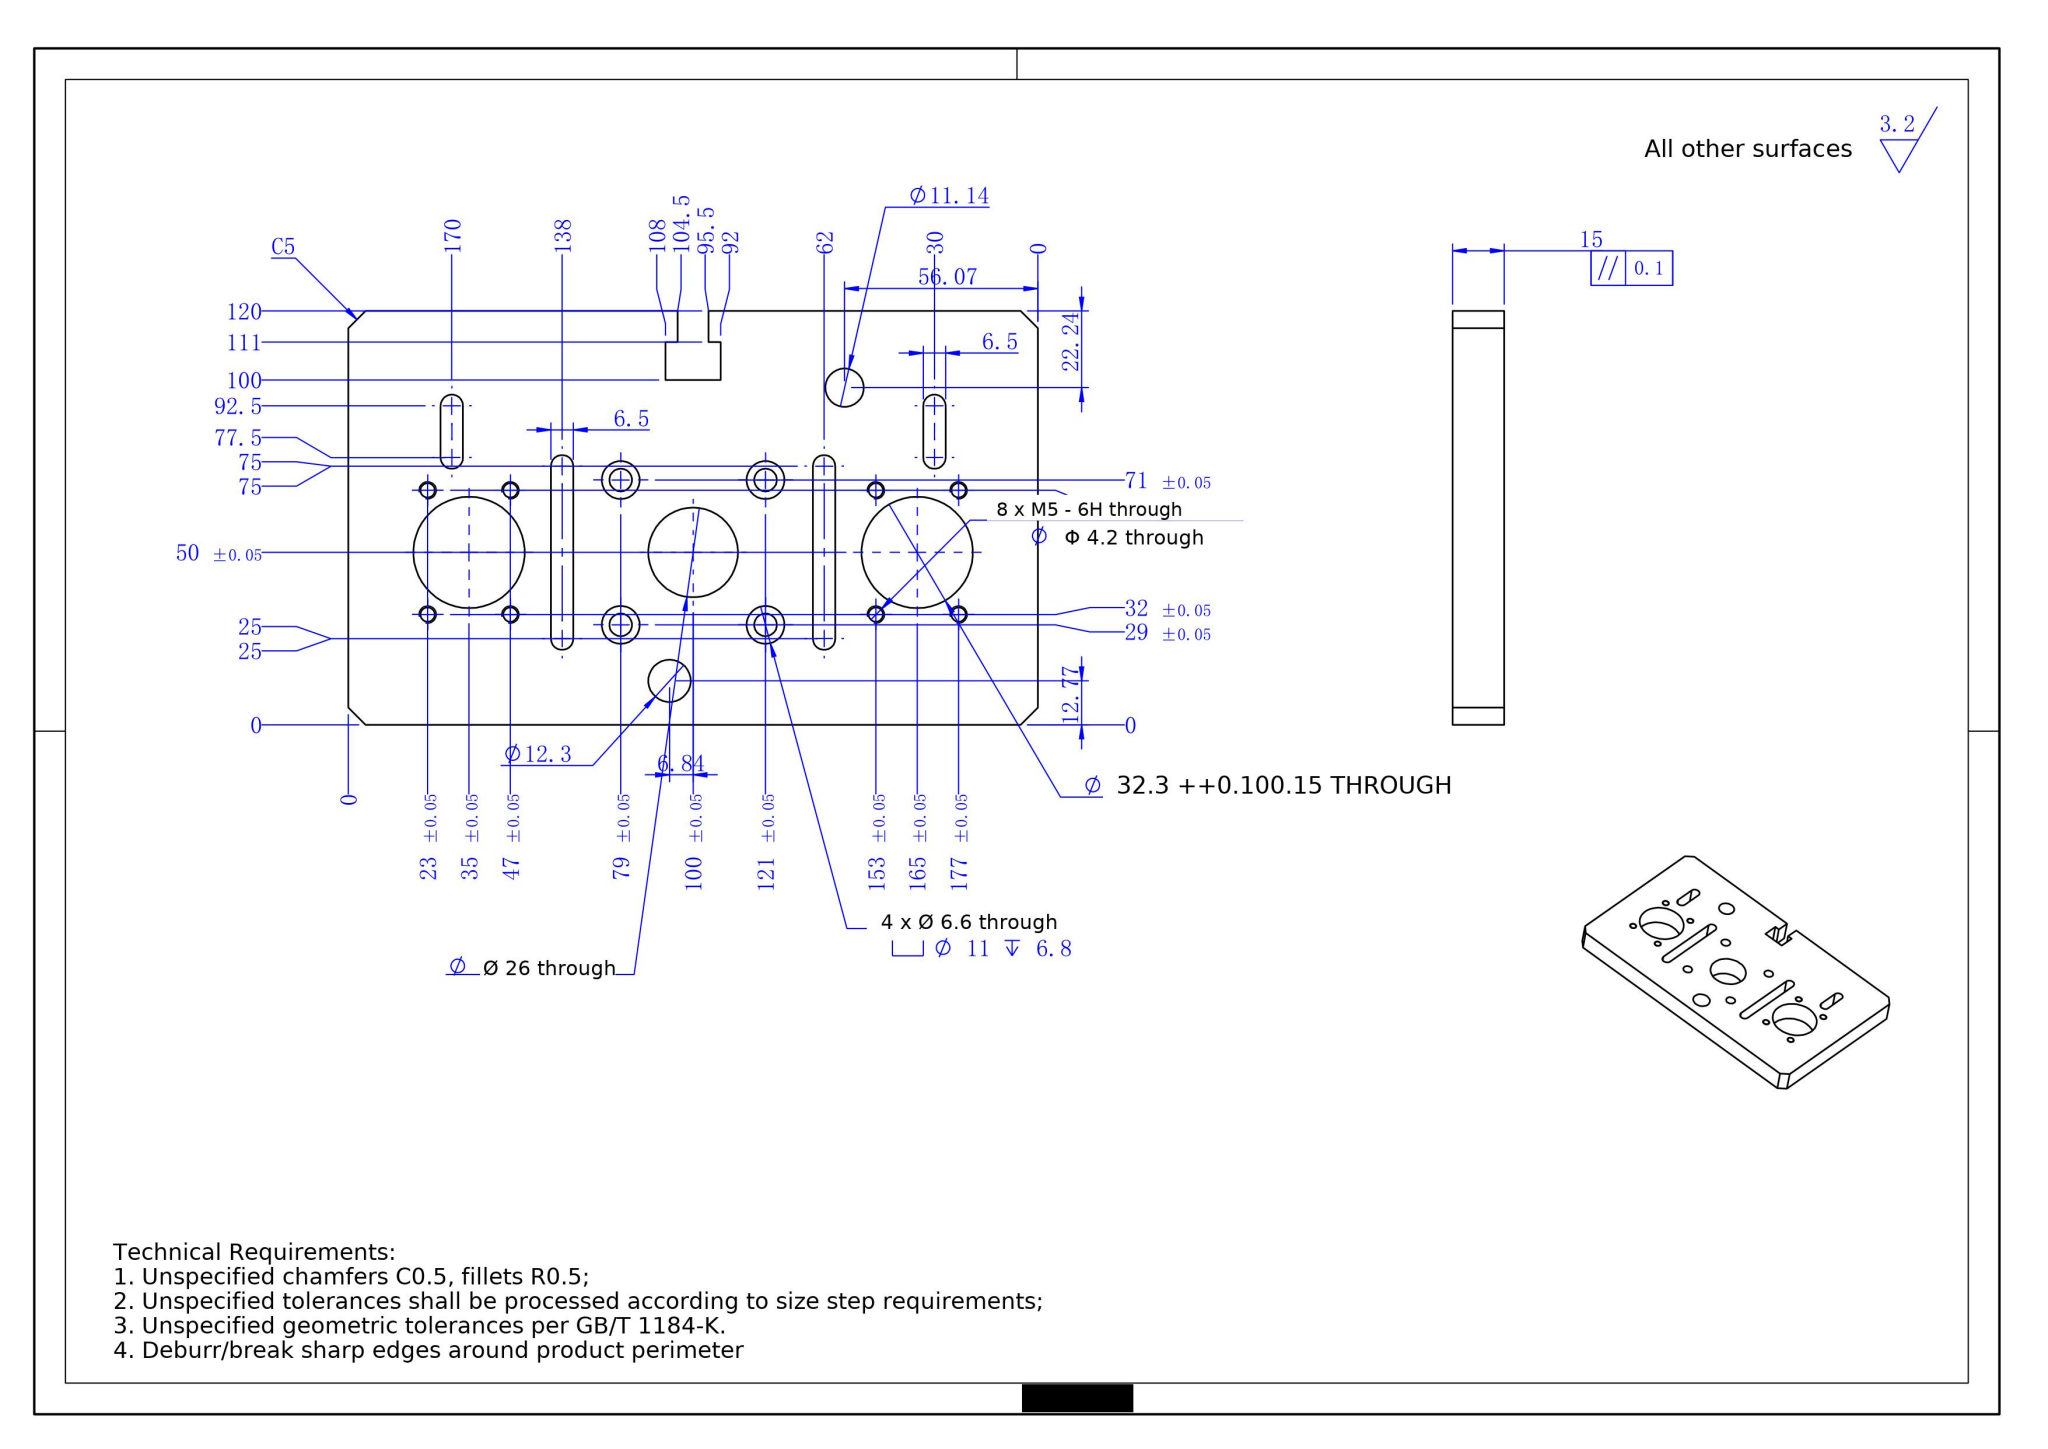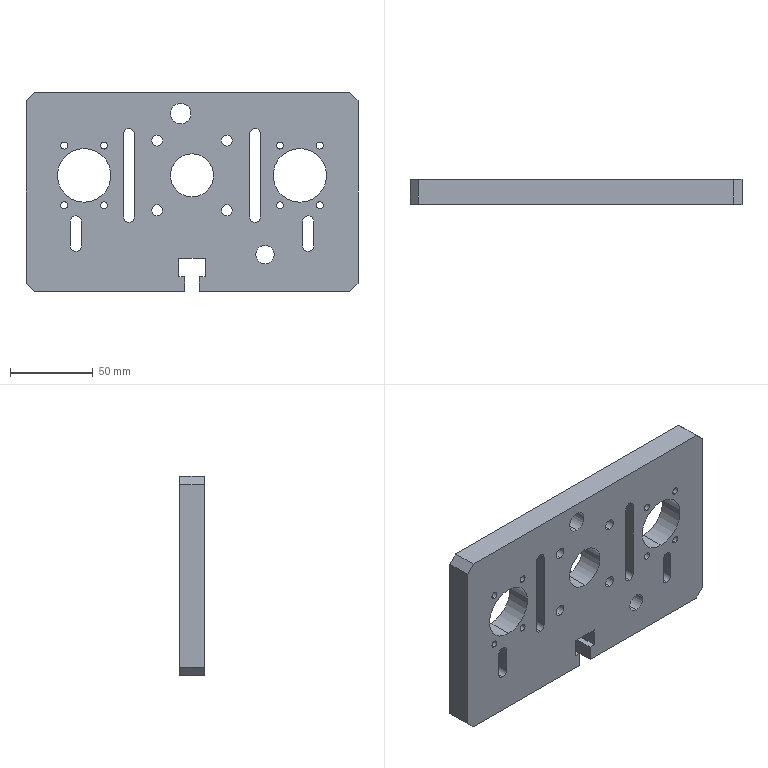Part | SolidWorks | mm | 1 solid | 84 faces | box 200 x 15 x 120 mm | volume 299568 mm3 | cylinder 54 | plane 30 | commonest cylinder face diameters 4.2 x16 6.5 x12 11 x8 6.6 x8 32.3 x4 12.3 x2 11.144 x2 26 x2
build123d program:
from build123d import *

# Parameters (mm, degrees)
SKETCH1_W                                          = 200
SKETCH1_H                                          = 120
BOSS_EXTRUDE1_DEPTH                                = 15
F_22_0_22_DIAMETER_HOLE1_D                         = 26
CUT_EXTRUDE2_DEPTH                                 = 15
SKETCH10_R                                         = 16.15
CUT_EXTRUDE3_DEPTH                                 = 165.165
HOLE_SIZE_ACCORDING_TO_TYPE_1_OF_HEXAG_D           = 6.6
HOLE_SIZE_ACCORDING_TO_TYPE_1_OF_HEXAG_CBORE_D     = 11
HOLE_SIZE_ACCORDING_TO_TYPE_1_OF_HEXAG_CBORE_DEPTH = 6.8
M5_TAPPED_HOLE1_D                                  = 4.2
CUT_EXTRUDE4_DEPTH                                 = 165.165
CUT_EXTRUDE5_DEPTH                                 = 165.165
CHAMFER1_SIZE                                      = 5
SKETCH17_R                                         = 6.15
SKETCH17_R_2                                       = 5.572
CUT_EXTRUDE6_DEPTH                                 = 80


with BuildPart() as part:
    # Sketch1 → Boss-Extrude1 (new body)
    with BuildSketch(Plane.XZ):
        with Locations((50, -5)):
            Rectangle(SKETCH1_W, SKETCH1_H)
    extrude(amount=-BOSS_EXTRUDE1_DEPTH)

    # 22.0 _22_ Diameter Hole1 (through all)
    with Locations(Plane(origin=(0, 0, 0), x_dir=(-1, 0, 0), z_dir=(0, -1, 0))):
        with Locations((-50, -5)):
            Hole(F_22_0_22_DIAMETER_HOLE1_D / 2)

    # Sketch9 → Cut-Extrude2 (cut)
    with BuildSketch(Plane(origin=(0, 15, 0), x_dir=(1, 0, 0), z_dir=(0, 1, 0))):
        Polygon((45.5, 56), (45.5, 65), (54.5, 65), (54.5, 56), (58, 56), (58, 45), (42, 45), (42, 56), align=None)
    extrude(amount=-CUT_EXTRUDE2_DEPTH, mode=Mode.SUBTRACT)

    # Sketch10 → Cut-Extrude3 (cut, through all)
    with BuildSketch(Plane.XZ):
        with Locations(Location((-15, 5, 0), (0, 0, 270))):
            Circle(SKETCH10_R)
        with Locations(Location((115, 5, 0), (0, 0, 270))):
            Circle(SKETCH10_R)
    extrude(amount=-CUT_EXTRUDE3_DEPTH, mode=Mode.SUBTRACT)

    # Hole Size _according to_ Type 1 of Hexag (through all)
    with Locations(Plane(origin=(0, 15, 0), x_dir=(1, 0, 0), z_dir=(0, 1, 0))):
        with Locations((71, 16), (29, 16), (29, -26), (71, -26)):
            CounterBoreHole(HOLE_SIZE_ACCORDING_TO_TYPE_1_OF_HEXAG_D / 2, HOLE_SIZE_ACCORDING_TO_TYPE_1_OF_HEXAG_CBORE_D / 2, HOLE_SIZE_ACCORDING_TO_TYPE_1_OF_HEXAG_CBORE_DEPTH)

    # M5 Tapped Hole1 (through all)
    with Locations(Plane(origin=(0, 0, 0), x_dir=(-1, 0, 0), z_dir=(0, -1, 0))):
        with Locations((27, -23), (3, -23), (3, 13), (27, 13), (-127, -23), (-103, -23), (-127, 13), (-103, 13)):
            Hole(M5_TAPPED_HOLE1_D / 2)

    # Sketch15 → Cut-Extrude4 (cut, through all)
    with BuildSketch(Plane.XZ):
        with BuildLine():
            Line((8.75, -20), (8.75, 30))
            ThreePointArc((8.75, 30), (12, 33.25), (15.25, 30))
            Line((15.25, 30), (15.25, -20))
            ThreePointArc((15.25, -20), (12, -23.25), (8.75, -20))
        make_face()
    cut_extrude4 = extrude(amount=-CUT_EXTRUDE4_DEPTH, mode=Mode.SUBTRACT)

    # Mirror2: Cut-Extrude4 across plane
    add(cut_extrude4.mirror(Plane.ZY.offset(-50)), mode=Mode.SUBTRACT)

    # Sketch16 → Cut-Extrude5 (cut, through all)
    with BuildSketch(Plane.XZ):
        with BuildLine():
            Line((-23.25, -37.5), (-23.25, -22.5))
            ThreePointArc((-23.25, -22.5), (-20, -19.25), (-16.75, -22.5))
            Line((-16.75, -22.5), (-16.75, -37.5))
            ThreePointArc((-16.75, -37.5), (-20, -40.75), (-23.25, -37.5))
        make_face()
        with BuildLine():
            Line((116.75, -37.5), (116.75, -22.5))
            ThreePointArc((116.75, -22.5), (120, -19.25), (123.25, -22.5))
            Line((123.25, -22.5), (123.25, -37.5))
            ThreePointArc((123.25, -37.5), (120, -40.75), (116.75, -37.5))
        make_face()
    extrude(amount=-CUT_EXTRUDE5_DEPTH, mode=Mode.SUBTRACT)

    # Chamfer1
    chamfer1_edges = [part.edges().sort_by_distance(p)[0] for p in [
        (-50, 7.5, 55),
        (150, 7.5, 55),
        (150, 7.5, -65),
        (-50, 7.5, -65),
    ]]
    chamfer(chamfer1_edges, length=CHAMFER1_SIZE)

    # Sketch17 → Cut-Extrude6 (cut)
    with BuildSketch(Plane(origin=(0, 0, 0), x_dir=(-1, 0, 0), z_dir=(0, -1, 0))):
        with Locations(Location((-43.156, -42.232, 0), (0, 0, 90))):
            Circle(SKETCH17_R)
        with Locations(Location((-93.933, 42.765, 0), (0, 0, 90))):
            Circle(SKETCH17_R_2)
    extrude(amount=-CUT_EXTRUDE6_DEPTH, mode=Mode.SUBTRACT)


solid = part.part